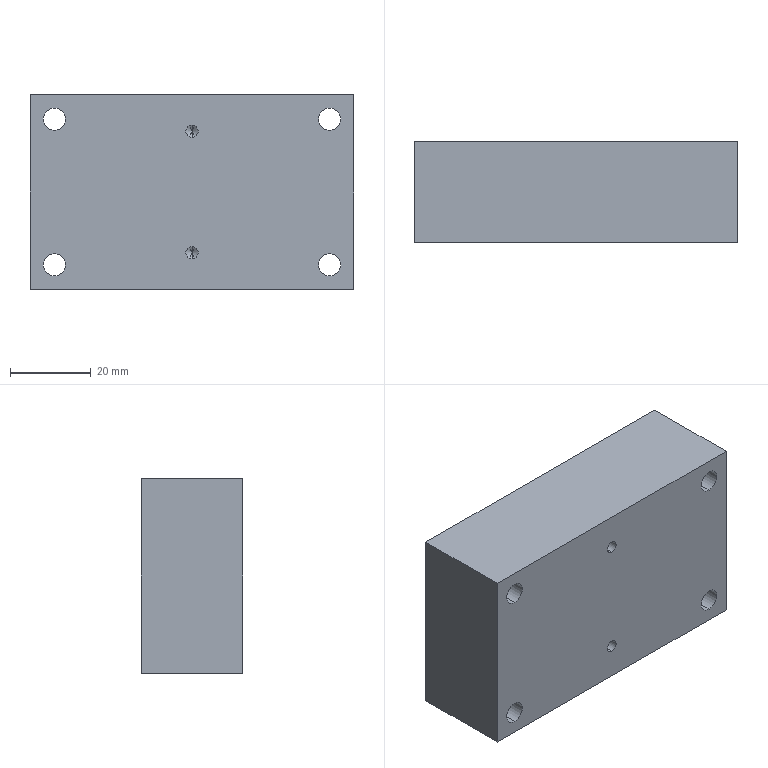Component | SolidWorks | F-YBExport-1-1_LSDH-6-027-1 | 1 solid | 42 faces | box 80 x 25 x 48 mm | volume 91100 mm3 | cylinder 24 | plane 10 | cone 8 | commonest cylinder face diameters 5.5 x8 10 x8 3 x4 2.5 x4
build123d program:
from build123d import *

# Parameters (mm, degrees)
SKETCH1_W                                            = 48
SKETCH1_H                                            = 80
BOSS_EXTRUDE1_DEPTH                                  = 25
SKETCH3_R                                            = 5
CUT_EXTRUDE1_DEPTH                                   = 5
HOLE_SIZE_ACCORDING_TO_HEX_SOCKET_HEAD_C_D           = 5.5
HOLE_SIZE_ACCORDING_TO_HEX_SOCKET_HEAD_C_CBORE_D     = 10
HOLE_SIZE_ACCORDING_TO_HEX_SOCKET_HEAD_C_CBORE_DEPTH = 5.7
M3_TAPPED_HOLE1_D                                    = 2.5
M3_TAPPED_HOLE1_DEPTH                                = 7.5
M3_TAPPED_HOLE1_TIP                                  = 0.7511
F_3_0_3_DIAMETER_HOLE1_D                             = 3
F_3_0_3_DIAMETER_HOLE1_DEPTH                         = 7
F_3_0_3_DIAMETER_HOLE1_TIP                           = 0.9013


with BuildPart() as part:
    # Sketch1 → Boss-Extrude1 (new body)
    with BuildSketch(Plane.XY):
        Rectangle(SKETCH1_W, SKETCH1_H)
    extrude(amount=BOSS_EXTRUDE1_DEPTH)

    # Sketch3 → Cut-Extrude1 (cut)
    with BuildSketch(Plane.XY.offset(25)):
        with Locations((-18, 34)):
            Circle(SKETCH3_R)
        with Locations((18, 34)):
            Circle(SKETCH3_R)
        with Locations((-18, -34)):
            Circle(SKETCH3_R)
        with Locations((18, -34)):
            Circle(SKETCH3_R)
    extrude(amount=-CUT_EXTRUDE1_DEPTH, mode=Mode.SUBTRACT)

    # Hole Size according to Hex Socket Head C (through all)
    with Locations(Plane(origin=(-18, 34, 20), x_dir=(1, 0, 0), z_dir=(0, 0, 1))):
        with Locations((0, 0), (36, 0), (36, -68), (0, -68)):
            CounterBoreHole(HOLE_SIZE_ACCORDING_TO_HEX_SOCKET_HEAD_C_D / 2, HOLE_SIZE_ACCORDING_TO_HEX_SOCKET_HEAD_C_CBORE_D / 2, HOLE_SIZE_ACCORDING_TO_HEX_SOCKET_HEAD_C_CBORE_DEPTH)

    # M3 Tapped Hole1
    with Locations(Plane(origin=(0, 10, 25), x_dir=(1, 0, 0), z_dir=(0, 0, 1))):
        with Locations((0, 0), (0, -30)):
            Hole(M3_TAPPED_HOLE1_D / 2, depth=M3_TAPPED_HOLE1_DEPTH)
            with Locations((0, 0, -(M3_TAPPED_HOLE1_DEPTH + M3_TAPPED_HOLE1_TIP / 2))):  # 118° drill point
                Cone(0, M3_TAPPED_HOLE1_D / 2, M3_TAPPED_HOLE1_TIP, mode=Mode.SUBTRACT)

    # 3.0 _3_ Diameter Hole1
    with Locations(Plane(origin=(15, 0, 0), x_dir=(-1, 0, 0), z_dir=(0, 0, -1))):
        with Locations((0, 0), (30, 0)):
            Hole(F_3_0_3_DIAMETER_HOLE1_D / 2, depth=F_3_0_3_DIAMETER_HOLE1_DEPTH)
            with Locations((0, 0, -(F_3_0_3_DIAMETER_HOLE1_DEPTH + F_3_0_3_DIAMETER_HOLE1_TIP / 2))):  # 118° drill point
                Cone(0, F_3_0_3_DIAMETER_HOLE1_D / 2, F_3_0_3_DIAMETER_HOLE1_TIP, mode=Mode.SUBTRACT)


solid = part.part

# Placed as in the assembly
solid = solid.moved(Location((329.305, 330.175, 175.979), (-90, 0, 90)))